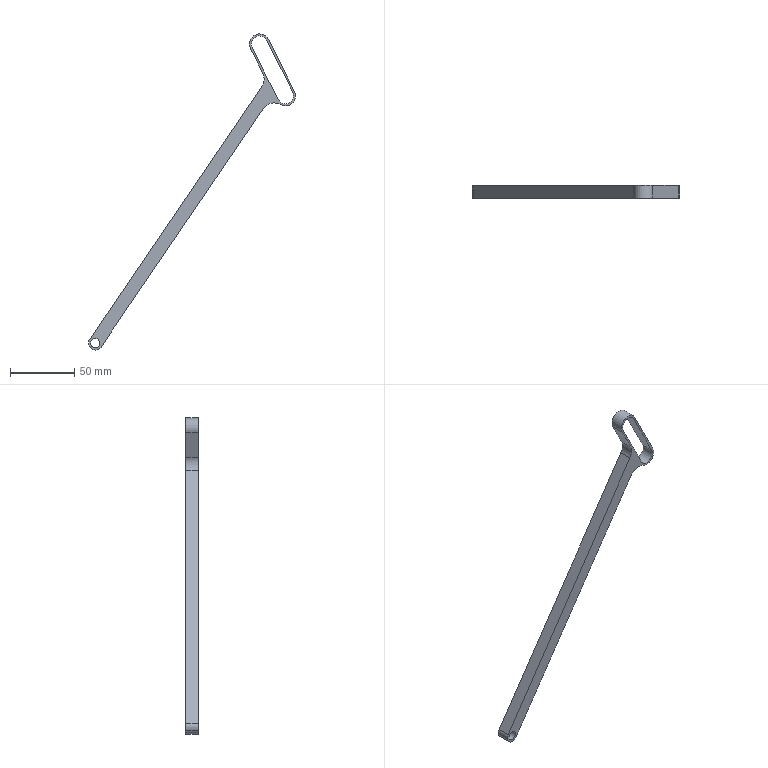Component | SolidWorks | Part1^LouverMechanism2-1 | 1 solid | 18 faces | box 161.29 x 10 x 246.24 mm | volume 28399 mm3 | cylinder 10 | plane 8 | commonest cylinder face diameters 7.233 x2 10.714 x2 15.803 x2 12.664 x2 20 x2
STEP:
#1=COLOUR_RGB('',0.7922,0.8196,0.9333);
#2=FILL_AREA_STYLE_COLOUR('',#1);
#3=FILL_AREA_STYLE('',(#2));
#4=SURFACE_STYLE_FILL_AREA(#3);
#5=SURFACE_SIDE_STYLE('',(#4));
#6=SURFACE_STYLE_USAGE(.BOTH.,#5);
#7=PRESENTATION_STYLE_ASSIGNMENT((#6));
#8=CARTESIAN_POINT('',(-4.368,20.955,35.082));
#9=VERTEX_POINT('',#8);
#10=CARTESIAN_POINT('',(-4.113,20.955,35.209));
#11=VERTEX_POINT('',#10);
#12=CARTESIAN_POINT('',(-4.241,20.955,35.145));
#13=DIRECTION('',(-0.,1.,-0.));
#14=DIRECTION('',(0.8942,0.,0.4477));
#15=AXIS2_PLACEMENT_3D('',#12,#13,#14);
#16=CIRCLE('',#15,0.1424);
#17=EDGE_CURVE('',#9,#11,#16,.T.);
#18=ORIENTED_EDGE('',*,*,#17,.T.);
#19=CARTESIAN_POINT('',(-4.113,20.561,35.209));
#20=VERTEX_POINT('',#19);
#21=CARTESIAN_POINT('',(-4.113,20.955,35.209));
#22=DIRECTION('',(0.,-1.,0.));
#23=VECTOR('',#22,39.37);
#24=LINE('',#21,#23);
#25=EDGE_CURVE('',#11,#20,#24,.T.);
#26=ORIENTED_EDGE('',*,*,#25,.T.);
#27=CARTESIAN_POINT('',(-4.368,20.561,35.082));
#28=VERTEX_POINT('',#27);
#29=CARTESIAN_POINT('',(-4.241,20.561,35.145));
#30=DIRECTION('',(-0.,1.,-0.));
#31=DIRECTION('',(0.8942,0.,0.4477));
#32=AXIS2_PLACEMENT_3D('',#29,#30,#31);
#33=CIRCLE('',#32,0.1424);
#34=EDGE_CURVE('',#28,#20,#33,.T.);
#35=ORIENTED_EDGE('',*,*,#34,.F.);
#36=CARTESIAN_POINT('',(-4.368,20.955,35.082));
#37=DIRECTION('',(0.,-1.,0.));
#38=VECTOR('',#37,39.37);
#39=LINE('',#36,#38);
#40=EDGE_CURVE('',#9,#28,#39,.T.);
#41=ORIENTED_EDGE('',*,*,#40,.F.);
#42=EDGE_LOOP('',(#18,#26,#35,#41));
#43=FACE_OUTER_BOUND('',#42,.T.);
#44=CARTESIAN_POINT('',(-4.241,20.955,35.145));
#45=DIRECTION('',(0.,-1.,0.));
#46=DIRECTION('',(-0.8942,0.,-0.4477));
#47=AXIS2_PLACEMENT_3D('',#44,#45,#46);
#48=CYLINDRICAL_SURFACE('',#47,0.1424);
#49=ADVANCED_FACE('',(#43),#48,.F.);
#50=CARTESIAN_POINT('',(-4.429,20.955,35.051));
#51=VERTEX_POINT('',#50);
#52=CARTESIAN_POINT('',(-4.415,20.955,35.264));
#53=VERTEX_POINT('',#52);
#54=CARTESIAN_POINT('',(-4.241,20.955,35.145));
#55=DIRECTION('',(-0.,1.,-0.));
#56=DIRECTION('',(0.8942,0.,0.4477));
#57=AXIS2_PLACEMENT_3D('',#54,#55,#56);
#58=CIRCLE('',#57,0.2109);
#59=EDGE_CURVE('',#51,#53,#58,.T.);
#60=ORIENTED_EDGE('',*,*,#59,.F.);
#61=CARTESIAN_POINT('',(-4.429,20.561,35.051));
#62=VERTEX_POINT('',#61);
#63=CARTESIAN_POINT('',(-4.429,20.955,35.051));
#64=DIRECTION('',(0.,-1.,0.));
#65=VECTOR('',#64,39.37);
#66=LINE('',#63,#65);
#67=EDGE_CURVE('',#51,#62,#66,.T.);
#68=ORIENTED_EDGE('',*,*,#67,.T.);
#69=CARTESIAN_POINT('',(-4.415,20.561,35.264));
#70=VERTEX_POINT('',#69);
#71=CARTESIAN_POINT('',(-4.241,20.561,35.145));
#72=DIRECTION('',(-0.,1.,-0.));
#73=DIRECTION('',(0.8942,0.,0.4477));
#74=AXIS2_PLACEMENT_3D('',#71,#72,#73);
#75=CIRCLE('',#74,0.2109);
#76=EDGE_CURVE('',#62,#70,#75,.T.);
#77=ORIENTED_EDGE('',*,*,#76,.T.);
#78=CARTESIAN_POINT('',(-4.415,20.955,35.264));
#79=DIRECTION('',(0.,-1.,0.));
#80=VECTOR('',#79,39.37);
#81=LINE('',#78,#80);
#82=EDGE_CURVE('',#53,#70,#81,.T.);
#83=ORIENTED_EDGE('',*,*,#82,.F.);
#84=EDGE_LOOP('',(#60,#68,#77,#83));
#85=FACE_OUTER_BOUND('',#84,.T.);
#86=CARTESIAN_POINT('',(-4.241,20.955,35.145));
#87=DIRECTION('',(0.,-1.,0.));
#88=DIRECTION('',(-0.8942,0.,-0.4477));
#89=AXIS2_PLACEMENT_3D('',#86,#87,#88);
#90=CYLINDRICAL_SURFACE('',#89,0.2109);
#91=ADVANCED_FACE('',(#85),#90,.T.);
#92=CARTESIAN_POINT('',(1.866,20.955,42.873));
#93=VERTEX_POINT('',#92);
#94=CARTESIAN_POINT('',(1.434,20.955,42.463));
#95=VERTEX_POINT('',#94);
#96=CARTESIAN_POINT('',(1.587,20.955,42.733));
#97=DIRECTION('',(-0.,1.,-0.));
#98=DIRECTION('',(0.8942,0.,0.4477));
#99=AXIS2_PLACEMENT_3D('',#96,#97,#98);
#100=CIRCLE('',#99,0.3111);
#101=EDGE_CURVE('',#93,#95,#100,.T.);
#102=ORIENTED_EDGE('',*,*,#101,.T.);
#103=CARTESIAN_POINT('',(0.9134,20.955,42.342));
#104=VERTEX_POINT('',#103);
#105=CARTESIAN_POINT('',(1.239,20.955,42.121));
#106=DIRECTION('',(0.,-1.,0.));
#107=DIRECTION('',(0.8942,0.,0.4477));
#108=AXIS2_PLACEMENT_3D('',#105,#106,#107);
#109=CIRCLE('',#108,0.3937);
#110=EDGE_CURVE('',#95,#104,#109,.T.);
#111=ORIENTED_EDGE('',*,*,#110,.T.);
#112=CARTESIAN_POINT('',(-4.066,20.955,35.027));
#113=VERTEX_POINT('',#112);
#114=CARTESIAN_POINT('',(1.214,20.955,42.784));
#115=DIRECTION('',(-0.5627,-0.,-0.8267));
#116=VECTOR('',#115,39.37);
#117=LINE('',#114,#116);
#118=EDGE_CURVE('',#104,#113,#117,.T.);
#119=ORIENTED_EDGE('',*,*,#118,.T.);
#120=CARTESIAN_POINT('',(-4.241,20.955,35.145));
#121=DIRECTION('',(-0.,1.,-0.));
#122=DIRECTION('',(0.8942,0.,0.4477));
#123=AXIS2_PLACEMENT_3D('',#120,#121,#122);
#124=CIRCLE('',#123,0.2109);
#125=EDGE_CURVE('',#113,#51,#124,.T.);
#126=ORIENTED_EDGE('',*,*,#125,.T.);
#127=ORIENTED_EDGE('',*,*,#59,.T.);
#128=CARTESIAN_POINT('',(0.8678,20.955,43.025));
#129=VERTEX_POINT('',#128);
#130=CARTESIAN_POINT('',(0.9756,20.955,43.183));
#131=DIRECTION('',(0.5627,0.,0.8267));
#132=VECTOR('',#131,39.37);
#133=LINE('',#130,#132);
#134=EDGE_CURVE('',#53,#129,#133,.T.);
#135=ORIENTED_EDGE('',*,*,#134,.T.);
#136=CARTESIAN_POINT('',(0.8944,20.955,43.423));
#137=VERTEX_POINT('',#136);
#138=CARTESIAN_POINT('',(0.5424,20.955,43.247));
#139=DIRECTION('',(0.,-1.,0.));
#140=DIRECTION('',(0.8942,0.,0.4477));
#141=AXIS2_PLACEMENT_3D('',#138,#139,#140);
#142=CIRCLE('',#141,0.3937);
#143=EDGE_CURVE('',#129,#137,#142,.T.);
#144=ORIENTED_EDGE('',*,*,#143,.T.);
#145=CARTESIAN_POINT('',(0.5162,20.955,44.178));
#146=VERTEX_POINT('',#145);
#147=CARTESIAN_POINT('',(0.9996,20.955,43.213));
#148=DIRECTION('',(-0.4477,0.,0.8942));
#149=VECTOR('',#148,39.37);
#150=LINE('',#147,#149);
#151=EDGE_CURVE('',#137,#146,#150,.T.);
#152=ORIENTED_EDGE('',*,*,#151,.T.);
#153=CARTESIAN_POINT('',(1.073,20.955,44.457));
#154=VERTEX_POINT('',#153);
#155=CARTESIAN_POINT('',(0.7943,20.955,44.318));
#156=DIRECTION('',(-0.,1.,-0.));
#157=DIRECTION('',(0.8942,0.,0.4477));
#158=AXIS2_PLACEMENT_3D('',#155,#156,#157);
#159=CIRCLE('',#158,0.3111);
#160=EDGE_CURVE('',#146,#154,#159,.T.);
#161=ORIENTED_EDGE('',*,*,#160,.T.);
#162=CARTESIAN_POINT('',(1.866,20.955,42.873));
#163=DIRECTION('',(0.4477,-0.,-0.8942));
#164=VECTOR('',#163,39.37);
#165=LINE('',#162,#164);
#166=EDGE_CURVE('',#154,#93,#165,.T.);
#167=ORIENTED_EDGE('',*,*,#166,.T.);
#168=EDGE_LOOP('',(#102,#111,#119,#126,#127,#135,#144,#152,#161,#167));
#169=FACE_OUTER_BOUND('',#168,.T.);
#170=ORIENTED_EDGE('',*,*,#17,.F.);
#171=CARTESIAN_POINT('',(-4.241,20.955,35.145));
#172=DIRECTION('',(-0.,1.,-0.));
#173=DIRECTION('',(0.8942,0.,0.4477));
#174=AXIS2_PLACEMENT_3D('',#171,#172,#173);
#175=CIRCLE('',#174,0.1424);
#176=EDGE_CURVE('',#11,#9,#175,.T.);
#177=ORIENTED_EDGE('',*,*,#176,.F.);
#178=EDGE_LOOP('',(#170,#177));
#179=FACE_BOUND('',#178,.T.);
#180=CARTESIAN_POINT('',(1.365,20.955,42.622));
#181=VERTEX_POINT('',#180);
#182=CARTESIAN_POINT('',(0.5714,20.955,44.206));
#183=VERTEX_POINT('',#182);
#184=CARTESIAN_POINT('',(1.365,20.955,42.622));
#185=DIRECTION('',(-0.4477,0.,0.8942));
#186=VECTOR('',#185,39.37);
#187=LINE('',#184,#186);
#188=EDGE_CURVE('',#181,#183,#187,.T.);
#189=ORIENTED_EDGE('',*,*,#188,.F.);
#190=CARTESIAN_POINT('',(1.81,20.955,42.845));
#191=VERTEX_POINT('',#190);
#192=CARTESIAN_POINT('',(1.587,20.955,42.733));
#193=DIRECTION('',(-0.,1.,-0.));
#194=DIRECTION('',(0.8942,0.,0.4477));
#195=AXIS2_PLACEMENT_3D('',#192,#193,#194);
#196=CIRCLE('',#195,0.2493);
#197=EDGE_CURVE('',#191,#181,#196,.T.);
#198=ORIENTED_EDGE('',*,*,#197,.F.);
#199=CARTESIAN_POINT('',(1.017,20.955,44.429));
#200=VERTEX_POINT('',#199);
#201=CARTESIAN_POINT('',(1.81,20.955,42.845));
#202=DIRECTION('',(0.4477,-0.,-0.8942));
#203=VECTOR('',#202,39.37);
#204=LINE('',#201,#203);
#205=EDGE_CURVE('',#200,#191,#204,.T.);
#206=ORIENTED_EDGE('',*,*,#205,.F.);
#207=CARTESIAN_POINT('',(0.7943,20.955,44.318));
#208=DIRECTION('',(-0.,1.,-0.));
#209=DIRECTION('',(0.8942,0.,0.4477));
#210=AXIS2_PLACEMENT_3D('',#207,#208,#209);
#211=CIRCLE('',#210,0.2493);
#212=EDGE_CURVE('',#183,#200,#211,.T.);
#213=ORIENTED_EDGE('',*,*,#212,.F.);
#214=EDGE_LOOP('',(#189,#198,#206,#213));
#215=FACE_BOUND('',#214,.T.);
#216=CARTESIAN_POINT('',(1.587,20.955,42.733));
#217=DIRECTION('',(-0.,1.,-0.));
#218=DIRECTION('',(0.8942,0.,0.4477));
#219=AXIS2_PLACEMENT_3D('',#216,#217,#218);
#220=PLANE('',#219);
#221=ADVANCED_FACE('',(#169,#179,#215),#220,.T.);
#222=ORIENTED_EDGE('',*,*,#34,.T.);
#223=CARTESIAN_POINT('',(-4.241,20.561,35.145));
#224=DIRECTION('',(-0.,1.,-0.));
#225=DIRECTION('',(0.8942,0.,0.4477));
#226=AXIS2_PLACEMENT_3D('',#223,#224,#225);
#227=CIRCLE('',#226,0.1424);
#228=EDGE_CURVE('',#20,#28,#227,.T.);
#229=ORIENTED_EDGE('',*,*,#228,.T.);
#230=EDGE_LOOP('',(#222,#229));
#231=FACE_BOUND('',#230,.T.);
#232=CARTESIAN_POINT('',(1.866,20.561,42.873));
#233=VERTEX_POINT('',#232);
#234=CARTESIAN_POINT('',(1.434,20.561,42.463));
#235=VERTEX_POINT('',#234);
#236=CARTESIAN_POINT('',(1.587,20.561,42.733));
#237=DIRECTION('',(-0.,1.,-0.));
#238=DIRECTION('',(0.8942,0.,0.4477));
#239=AXIS2_PLACEMENT_3D('',#236,#237,#238);
#240=CIRCLE('',#239,0.3111);
#241=EDGE_CURVE('',#233,#235,#240,.T.);
#242=ORIENTED_EDGE('',*,*,#241,.F.);
#243=CARTESIAN_POINT('',(1.073,20.561,44.457));
#244=VERTEX_POINT('',#243);
#245=CARTESIAN_POINT('',(1.866,20.561,42.873));
#246=DIRECTION('',(0.4477,-0.,-0.8942));
#247=VECTOR('',#246,39.37);
#248=LINE('',#245,#247);
#249=EDGE_CURVE('',#244,#233,#248,.T.);
#250=ORIENTED_EDGE('',*,*,#249,.F.);
#251=CARTESIAN_POINT('',(0.5162,20.561,44.178));
#252=VERTEX_POINT('',#251);
#253=CARTESIAN_POINT('',(0.7943,20.561,44.318));
#254=DIRECTION('',(-0.,1.,-0.));
#255=DIRECTION('',(0.8942,0.,0.4477));
#256=AXIS2_PLACEMENT_3D('',#253,#254,#255);
#257=CIRCLE('',#256,0.3111);
#258=EDGE_CURVE('',#252,#244,#257,.T.);
#259=ORIENTED_EDGE('',*,*,#258,.F.);
#260=CARTESIAN_POINT('',(0.8944,20.561,43.423));
#261=VERTEX_POINT('',#260);
#262=CARTESIAN_POINT('',(0.9996,20.561,43.213));
#263=DIRECTION('',(-0.4477,0.,0.8942));
#264=VECTOR('',#263,39.37);
#265=LINE('',#262,#264);
#266=EDGE_CURVE('',#261,#252,#265,.T.);
#267=ORIENTED_EDGE('',*,*,#266,.F.);
#268=CARTESIAN_POINT('',(0.8678,20.561,43.025));
#269=VERTEX_POINT('',#268);
#270=CARTESIAN_POINT('',(0.5424,20.561,43.247));
#271=DIRECTION('',(-0.,1.,-0.));
#272=DIRECTION('',(0.8942,0.,0.4477));
#273=AXIS2_PLACEMENT_3D('',#270,#271,#272);
#274=CIRCLE('',#273,0.3937);
#275=EDGE_CURVE('',#261,#269,#274,.T.);
#276=ORIENTED_EDGE('',*,*,#275,.T.);
#277=CARTESIAN_POINT('',(0.9756,20.561,43.183));
#278=DIRECTION('',(0.5627,0.,0.8267));
#279=VECTOR('',#278,39.37);
#280=LINE('',#277,#279);
#281=EDGE_CURVE('',#70,#269,#280,.T.);
#282=ORIENTED_EDGE('',*,*,#281,.F.);
#283=ORIENTED_EDGE('',*,*,#76,.F.);
#284=CARTESIAN_POINT('',(-4.066,20.561,35.027));
#285=VERTEX_POINT('',#284);
#286=CARTESIAN_POINT('',(-4.241,20.561,35.145));
#287=DIRECTION('',(-0.,1.,-0.));
#288=DIRECTION('',(0.8942,0.,0.4477));
#289=AXIS2_PLACEMENT_3D('',#286,#287,#288);
#290=CIRCLE('',#289,0.2109);
#291=EDGE_CURVE('',#285,#62,#290,.T.);
#292=ORIENTED_EDGE('',*,*,#291,.F.);
#293=CARTESIAN_POINT('',(0.9134,20.561,42.342));
#294=VERTEX_POINT('',#293);
#295=CARTESIAN_POINT('',(1.214,20.561,42.784));
#296=DIRECTION('',(-0.5627,-0.,-0.8267));
#297=VECTOR('',#296,39.37);
#298=LINE('',#295,#297);
#299=EDGE_CURVE('',#294,#285,#298,.T.);
#300=ORIENTED_EDGE('',*,*,#299,.F.);
#301=CARTESIAN_POINT('',(1.239,20.561,42.121));
#302=DIRECTION('',(-0.,1.,-0.));
#303=DIRECTION('',(0.8942,0.,0.4477));
#304=AXIS2_PLACEMENT_3D('',#301,#302,#303);
#305=CIRCLE('',#304,0.3937);
#306=EDGE_CURVE('',#294,#235,#305,.T.);
#307=ORIENTED_EDGE('',*,*,#306,.T.);
#308=EDGE_LOOP('',(#242,#250,#259,#267,#276,#282,#283,#292,#300,#307));
#309=FACE_OUTER_BOUND('',#308,.T.);
#310=CARTESIAN_POINT('',(1.81,20.561,42.845));
#311=VERTEX_POINT('',#310);
#312=CARTESIAN_POINT('',(1.365,20.561,42.622));
#313=VERTEX_POINT('',#312);
#314=CARTESIAN_POINT('',(1.587,20.561,42.733));
#315=DIRECTION('',(-0.,1.,-0.));
#316=DIRECTION('',(0.8942,0.,0.4477));
#317=AXIS2_PLACEMENT_3D('',#314,#315,#316);
#318=CIRCLE('',#317,0.2493);
#319=EDGE_CURVE('',#311,#313,#318,.T.);
#320=ORIENTED_EDGE('',*,*,#319,.T.);
#321=CARTESIAN_POINT('',(0.5714,20.561,44.206));
#322=VERTEX_POINT('',#321);
#323=CARTESIAN_POINT('',(1.365,20.561,42.622));
#324=DIRECTION('',(-0.4477,0.,0.8942));
#325=VECTOR('',#324,39.37);
#326=LINE('',#323,#325);
#327=EDGE_CURVE('',#313,#322,#326,.T.);
#328=ORIENTED_EDGE('',*,*,#327,.T.);
#329=CARTESIAN_POINT('',(1.017,20.561,44.429));
#330=VERTEX_POINT('',#329);
#331=CARTESIAN_POINT('',(0.7943,20.561,44.318));
#332=DIRECTION('',(-0.,1.,-0.));
#333=DIRECTION('',(0.8942,0.,0.4477));
#334=AXIS2_PLACEMENT_3D('',#331,#332,#333);
#335=CIRCLE('',#334,0.2493);
#336=EDGE_CURVE('',#322,#330,#335,.T.);
#337=ORIENTED_EDGE('',*,*,#336,.T.);
#338=CARTESIAN_POINT('',(1.81,20.561,42.845));
#339=DIRECTION('',(0.4477,-0.,-0.8942));
#340=VECTOR('',#339,39.37);
#341=LINE('',#338,#340);
#342=EDGE_CURVE('',#330,#311,#341,.T.);
#343=ORIENTED_EDGE('',*,*,#342,.T.);
#344=EDGE_LOOP('',(#320,#328,#337,#343));
#345=FACE_BOUND('',#344,.T.);
#346=CARTESIAN_POINT('',(1.587,20.561,42.733));
#347=DIRECTION('',(-0.,1.,-0.));
#348=DIRECTION('',(0.8942,0.,0.4477));
#349=AXIS2_PLACEMENT_3D('',#346,#347,#348);
#350=PLANE('',#349);
#351=ADVANCED_FACE('',(#231,#309,#345),#350,.F.);
#352=ORIENTED_EDGE('',*,*,#241,.T.);
#353=CARTESIAN_POINT('',(1.434,20.955,42.463));
#354=DIRECTION('',(-0.,1.,-0.));
#355=VECTOR('',#354,39.37);
#356=LINE('',#353,#355);
#357=EDGE_CURVE('',#235,#95,#356,.T.);
#358=ORIENTED_EDGE('',*,*,#357,.T.);
#359=ORIENTED_EDGE('',*,*,#101,.F.);
#360=CARTESIAN_POINT('',(1.866,20.955,42.873));
#361=DIRECTION('',(0.,-1.,0.));
#362=VECTOR('',#361,39.37);
#363=LINE('',#360,#362);
#364=EDGE_CURVE('',#93,#233,#363,.T.);
#365=ORIENTED_EDGE('',*,*,#364,.T.);
#366=EDGE_LOOP('',(#352,#358,#359,#365));
#367=FACE_OUTER_BOUND('',#366,.T.);
#368=CARTESIAN_POINT('',(1.587,20.955,42.733));
#369=DIRECTION('',(0.,-1.,0.));
#370=DIRECTION('',(-0.8942,0.,-0.4477));
#371=AXIS2_PLACEMENT_3D('',#368,#369,#370);
#372=CYLINDRICAL_SURFACE('',#371,0.3111);
#373=ADVANCED_FACE('',(#367),#372,.T.);
#374=ORIENTED_EDGE('',*,*,#118,.F.);
#375=CARTESIAN_POINT('',(0.9134,20.561,42.342));
#376=DIRECTION('',(0.,-1.,0.));
#377=VECTOR('',#376,39.37);
#378=LINE('',#375,#377);
#379=EDGE_CURVE('',#104,#294,#378,.T.);
#380=ORIENTED_EDGE('',*,*,#379,.T.);
#381=ORIENTED_EDGE('',*,*,#299,.T.);
#382=CARTESIAN_POINT('',(-4.066,20.955,35.027));
#383=DIRECTION('',(0.,-1.,0.));
#384=VECTOR('',#383,39.37);
#385=LINE('',#382,#384);
#386=EDGE_CURVE('',#113,#285,#385,.T.);
#387=ORIENTED_EDGE('',*,*,#386,.F.);
#388=EDGE_LOOP('',(#374,#380,#381,#387));
#389=FACE_OUTER_BOUND('',#388,.T.);
#390=CARTESIAN_POINT('',(1.214,20.955,42.784));
#391=DIRECTION('',(-0.8267,0.,0.5627));
#392=DIRECTION('',(0.5627,0.,0.8267));
#393=AXIS2_PLACEMENT_3D('',#390,#391,#392);
#394=PLANE('',#393);
#395=ADVANCED_FACE('',(#389),#394,.F.);
#396=ORIENTED_EDGE('',*,*,#67,.F.);
#397=ORIENTED_EDGE('',*,*,#125,.F.);
#398=ORIENTED_EDGE('',*,*,#386,.T.);
#399=ORIENTED_EDGE('',*,*,#291,.T.);
#400=EDGE_LOOP('',(#396,#397,#398,#399));
#401=FACE_OUTER_BOUND('',#400,.T.);
#402=CARTESIAN_POINT('',(-4.241,20.955,35.145));
#403=DIRECTION('',(0.,-1.,0.));
#404=DIRECTION('',(-0.8942,0.,-0.4477));
#405=AXIS2_PLACEMENT_3D('',#402,#403,#404);
#406=CYLINDRICAL_SURFACE('',#405,0.2109);
#407=ADVANCED_FACE('',(#401),#406,.T.);
#408=ORIENTED_EDGE('',*,*,#281,.T.);
#409=CARTESIAN_POINT('',(0.8678,20.955,43.025));
#410=DIRECTION('',(-0.,1.,-0.));
#411=VECTOR('',#410,39.37);
#412=LINE('',#409,#411);
#413=EDGE_CURVE('',#269,#129,#412,.T.);
#414=ORIENTED_EDGE('',*,*,#413,.T.);
#415=ORIENTED_EDGE('',*,*,#134,.F.);
#416=ORIENTED_EDGE('',*,*,#82,.T.);
#417=EDGE_LOOP('',(#408,#414,#415,#416));
#418=FACE_OUTER_BOUND('',#417,.T.);
#419=CARTESIAN_POINT('',(0.9756,20.955,43.183));
#420=DIRECTION('',(0.8267,-0.,-0.5627));
#421=DIRECTION('',(-0.5627,-0.,-0.8267));
#422=AXIS2_PLACEMENT_3D('',#419,#420,#421);
#423=PLANE('',#422);
#424=ADVANCED_FACE('',(#418),#423,.F.);
#425=ORIENTED_EDGE('',*,*,#151,.F.);
#426=CARTESIAN_POINT('',(0.8944,20.561,43.423));
#427=DIRECTION('',(0.,-1.,0.));
#428=VECTOR('',#427,39.37);
#429=LINE('',#426,#428);
#430=EDGE_CURVE('',#137,#261,#429,.T.);
#431=ORIENTED_EDGE('',*,*,#430,.T.);
#432=ORIENTED_EDGE('',*,*,#266,.T.);
#433=CARTESIAN_POINT('',(0.5162,20.955,44.178));
#434=DIRECTION('',(0.,-1.,0.));
#435=VECTOR('',#434,39.37);
#436=LINE('',#433,#435);
#437=EDGE_CURVE('',#146,#252,#436,.T.);
#438=ORIENTED_EDGE('',*,*,#437,.F.);
#439=EDGE_LOOP('',(#425,#431,#432,#438));
#440=FACE_OUTER_BOUND('',#439,.T.);
#441=CARTESIAN_POINT('',(0.9996,20.955,43.213));
#442=DIRECTION('',(0.8942,0.,0.4477));
#443=DIRECTION('',(0.,-1.,0.));
#444=AXIS2_PLACEMENT_3D('',#441,#442,#443);
#445=PLANE('',#444);
#446=ADVANCED_FACE('',(#440),#445,.F.);
#447=ORIENTED_EDGE('',*,*,#258,.T.);
#448=CARTESIAN_POINT('',(1.073,20.955,44.457));
#449=DIRECTION('',(0.,-1.,0.));
#450=VECTOR('',#449,39.37);
#451=LINE('',#448,#450);
#452=EDGE_CURVE('',#154,#244,#451,.T.);
#453=ORIENTED_EDGE('',*,*,#452,.F.);
#454=ORIENTED_EDGE('',*,*,#160,.F.);
#455=ORIENTED_EDGE('',*,*,#437,.T.);
#456=EDGE_LOOP('',(#447,#453,#454,#455));
#457=FACE_OUTER_BOUND('',#456,.T.);
#458=CARTESIAN_POINT('',(0.7943,20.955,44.318));
#459=DIRECTION('',(0.,-1.,0.));
#460=DIRECTION('',(-0.8942,0.,-0.4477));
#461=AXIS2_PLACEMENT_3D('',#458,#459,#460);
#462=CYLINDRICAL_SURFACE('',#461,0.3111);
#463=ADVANCED_FACE('',(#457),#462,.T.);
#464=ORIENTED_EDGE('',*,*,#249,.T.);
#465=ORIENTED_EDGE('',*,*,#364,.F.);
#466=ORIENTED_EDGE('',*,*,#166,.F.);
#467=ORIENTED_EDGE('',*,*,#452,.T.);
#468=EDGE_LOOP('',(#464,#465,#466,#467));
#469=FACE_OUTER_BOUND('',#468,.T.);
#470=CARTESIAN_POINT('',(1.866,20.955,42.873));
#471=DIRECTION('',(-0.8942,-0.,-0.4477));
#472=DIRECTION('',(-0.4477,0.,0.8942));
#473=AXIS2_PLACEMENT_3D('',#470,#471,#472);
#474=PLANE('',#473);
#475=ADVANCED_FACE('',(#469),#474,.F.);
#476=ORIENTED_EDGE('',*,*,#25,.F.);
#477=ORIENTED_EDGE('',*,*,#176,.T.);
#478=ORIENTED_EDGE('',*,*,#40,.T.);
#479=ORIENTED_EDGE('',*,*,#228,.F.);
#480=EDGE_LOOP('',(#476,#477,#478,#479));
#481=FACE_OUTER_BOUND('',#480,.T.);
#482=CARTESIAN_POINT('',(-4.241,20.955,35.145));
#483=DIRECTION('',(0.,-1.,0.));
#484=DIRECTION('',(-0.8942,0.,-0.4477));
#485=AXIS2_PLACEMENT_3D('',#482,#483,#484);
#486=CYLINDRICAL_SURFACE('',#485,0.1424);
#487=ADVANCED_FACE('',(#481),#486,.F.);
#488=ORIENTED_EDGE('',*,*,#319,.F.);
#489=CARTESIAN_POINT('',(1.81,20.955,42.845));
#490=DIRECTION('',(0.,-1.,0.));
#491=VECTOR('',#490,39.37);
#492=LINE('',#489,#491);
#493=EDGE_CURVE('',#191,#311,#492,.T.);
#494=ORIENTED_EDGE('',*,*,#493,.F.);
#495=ORIENTED_EDGE('',*,*,#197,.T.);
#496=CARTESIAN_POINT('',(1.365,20.955,42.622));
#497=DIRECTION('',(0.,-1.,0.));
#498=VECTOR('',#497,39.37);
#499=LINE('',#496,#498);
#500=EDGE_CURVE('',#181,#313,#499,.T.);
#501=ORIENTED_EDGE('',*,*,#500,.T.);
#502=EDGE_LOOP('',(#488,#494,#495,#501));
#503=FACE_OUTER_BOUND('',#502,.T.);
#504=CARTESIAN_POINT('',(1.587,20.955,42.733));
#505=DIRECTION('',(0.,-1.,0.));
#506=DIRECTION('',(-0.8942,0.,-0.4477));
#507=AXIS2_PLACEMENT_3D('',#504,#505,#506);
#508=CYLINDRICAL_SURFACE('',#507,0.2493);
#509=ADVANCED_FACE('',(#503),#508,.F.);
#510=ORIENTED_EDGE('',*,*,#327,.F.);
#511=ORIENTED_EDGE('',*,*,#500,.F.);
#512=ORIENTED_EDGE('',*,*,#188,.T.);
#513=CARTESIAN_POINT('',(0.5714,20.955,44.206));
#514=DIRECTION('',(0.,-1.,0.));
#515=VECTOR('',#514,39.37);
#516=LINE('',#513,#515);
#517=EDGE_CURVE('',#183,#322,#516,.T.);
#518=ORIENTED_EDGE('',*,*,#517,.T.);
#519=EDGE_LOOP('',(#510,#511,#512,#518));
#520=FACE_OUTER_BOUND('',#519,.T.);
#521=CARTESIAN_POINT('',(1.365,20.955,42.622));
#522=DIRECTION('',(0.8942,0.,0.4477));
#523=DIRECTION('',(0.,-1.,0.));
#524=AXIS2_PLACEMENT_3D('',#521,#522,#523);
#525=PLANE('',#524);
#526=ADVANCED_FACE('',(#520),#525,.T.);
#527=ORIENTED_EDGE('',*,*,#336,.F.);
#528=ORIENTED_EDGE('',*,*,#517,.F.);
#529=ORIENTED_EDGE('',*,*,#212,.T.);
#530=CARTESIAN_POINT('',(1.017,20.955,44.429));
#531=DIRECTION('',(0.,-1.,0.));
#532=VECTOR('',#531,39.37);
#533=LINE('',#530,#532);
#534=EDGE_CURVE('',#200,#330,#533,.T.);
#535=ORIENTED_EDGE('',*,*,#534,.T.);
#536=EDGE_LOOP('',(#527,#528,#529,#535));
#537=FACE_OUTER_BOUND('',#536,.T.);
#538=CARTESIAN_POINT('',(0.7943,20.955,44.318));
#539=DIRECTION('',(0.,-1.,0.));
#540=DIRECTION('',(-0.8942,0.,-0.4477));
#541=AXIS2_PLACEMENT_3D('',#538,#539,#540);
#542=CYLINDRICAL_SURFACE('',#541,0.2493);
#543=ADVANCED_FACE('',(#537),#542,.F.);
#544=ORIENTED_EDGE('',*,*,#342,.F.);
#545=ORIENTED_EDGE('',*,*,#534,.F.);
#546=ORIENTED_EDGE('',*,*,#205,.T.);
#547=ORIENTED_EDGE('',*,*,#493,.T.);
#548=EDGE_LOOP('',(#544,#545,#546,#547));
#549=FACE_OUTER_BOUND('',#548,.T.);
#550=CARTESIAN_POINT('',(1.81,20.955,42.845));
#551=DIRECTION('',(-0.8942,-0.,-0.4477));
#552=DIRECTION('',(-0.,1.,-0.));
#553=AXIS2_PLACEMENT_3D('',#550,#551,#552);
#554=PLANE('',#553);
#555=ADVANCED_FACE('',(#549),#554,.T.);
#556=ORIENTED_EDGE('',*,*,#143,.F.);
#557=ORIENTED_EDGE('',*,*,#413,.F.);
#558=ORIENTED_EDGE('',*,*,#275,.F.);
#559=ORIENTED_EDGE('',*,*,#430,.F.);
#560=EDGE_LOOP('',(#556,#557,#558,#559));
#561=FACE_OUTER_BOUND('',#560,.T.);
#562=CARTESIAN_POINT('',(0.5424,20.955,43.247));
#563=DIRECTION('',(-0.,1.,-0.));
#564=DIRECTION('',(0.8942,0.,0.4477));
#565=AXIS2_PLACEMENT_3D('',#562,#563,#564);
#566=CYLINDRICAL_SURFACE('',#565,0.3937);
#567=ADVANCED_FACE('',(#561),#566,.F.);
#568=ORIENTED_EDGE('',*,*,#110,.F.);
#569=ORIENTED_EDGE('',*,*,#357,.F.);
#570=ORIENTED_EDGE('',*,*,#306,.F.);
#571=ORIENTED_EDGE('',*,*,#379,.F.);
#572=EDGE_LOOP('',(#568,#569,#570,#571));
#573=FACE_OUTER_BOUND('',#572,.T.);
#574=CARTESIAN_POINT('',(1.239,20.955,42.121));
#575=DIRECTION('',(0.,-1.,0.));
#576=DIRECTION('',(-0.8942,0.,-0.4477));
#577=AXIS2_PLACEMENT_3D('',#574,#575,#576);
#578=CYLINDRICAL_SURFACE('',#577,0.3937);
#579=ADVANCED_FACE('',(#573),#578,.F.);
#580=CLOSED_SHELL('',(#49,#91,#221,#351,#373,#395,#407,#424,#446,#463,#475,#487,#509,#526,#543,#555,#567,#579));
#581=MANIFOLD_SOLID_BREP('',#580);
#582=STYLED_ITEM('',(#7),#581);
#583=(LENGTH_UNIT()NAMED_UNIT(*)SI_UNIT($,.METRE.));
#584=LENGTH_MEASURE_WITH_UNIT(LENGTH_MEASURE(0.0254),#583);
#585=DIMENSIONAL_EXPONENTS(1.,0.,0.,0.,0.,0.,0.);
#586=(CONVERSION_BASED_UNIT('',#584)LENGTH_UNIT()NAMED_UNIT(#585));
#587=UNCERTAINTY_MEASURE_WITH_UNIT(LENGTH_MEASURE(0.00001),#586,'','');
#588=(NAMED_UNIT(*)PLANE_ANGLE_UNIT()SI_UNIT($,.RADIAN.));
#589=(NAMED_UNIT(*)SI_UNIT($,.STERADIAN.)SOLID_ANGLE_UNIT());
#590=(GEOMETRIC_REPRESENTATION_CONTEXT(3)GLOBAL_UNCERTAINTY_ASSIGNED_CONTEXT((#587))GLOBAL_UNIT_ASSIGNED_CONTEXT((#586,#588,#589))REPRESENTATION_CONTEXT('',''));
#591=MECHANICAL_DESIGN_GEOMETRIC_PRESENTATION_REPRESENTATION('',(#582),#590);
#592=PRESENTATION_LAYER_ASSIGNMENT('','',(#582));
#593=CARTESIAN_POINT('',(0.,0.,0.));
#594=DIRECTION('',(0.,0.,1.));
#595=DIRECTION('',(1.,0.,0.));
#596=AXIS2_PLACEMENT_3D('',#593,#594,#595);
#597=(LENGTH_UNIT()NAMED_UNIT(*)SI_UNIT($,.METRE.));
#598=LENGTH_MEASURE_WITH_UNIT(LENGTH_MEASURE(0.0254),#597);
#599=DIMENSIONAL_EXPONENTS(1.,0.,0.,0.,0.,0.,0.);
#600=(CONVERSION_BASED_UNIT('',#598)LENGTH_UNIT()NAMED_UNIT(#599));
#601=UNCERTAINTY_MEASURE_WITH_UNIT(LENGTH_MEASURE(0.00001),#600,'','');
#602=(NAMED_UNIT(*)PLANE_ANGLE_UNIT()SI_UNIT($,.RADIAN.));
#603=(NAMED_UNIT(*)SI_UNIT($,.STERADIAN.)SOLID_ANGLE_UNIT());
#604=(GEOMETRIC_REPRESENTATION_CONTEXT(3)GLOBAL_UNCERTAINTY_ASSIGNED_CONTEXT((#601))GLOBAL_UNIT_ASSIGNED_CONTEXT((#600,#602,#603))REPRESENTATION_CONTEXT('',''));
#605=ADVANCED_BREP_SHAPE_REPRESENTATION('',(#581,#596),#604);